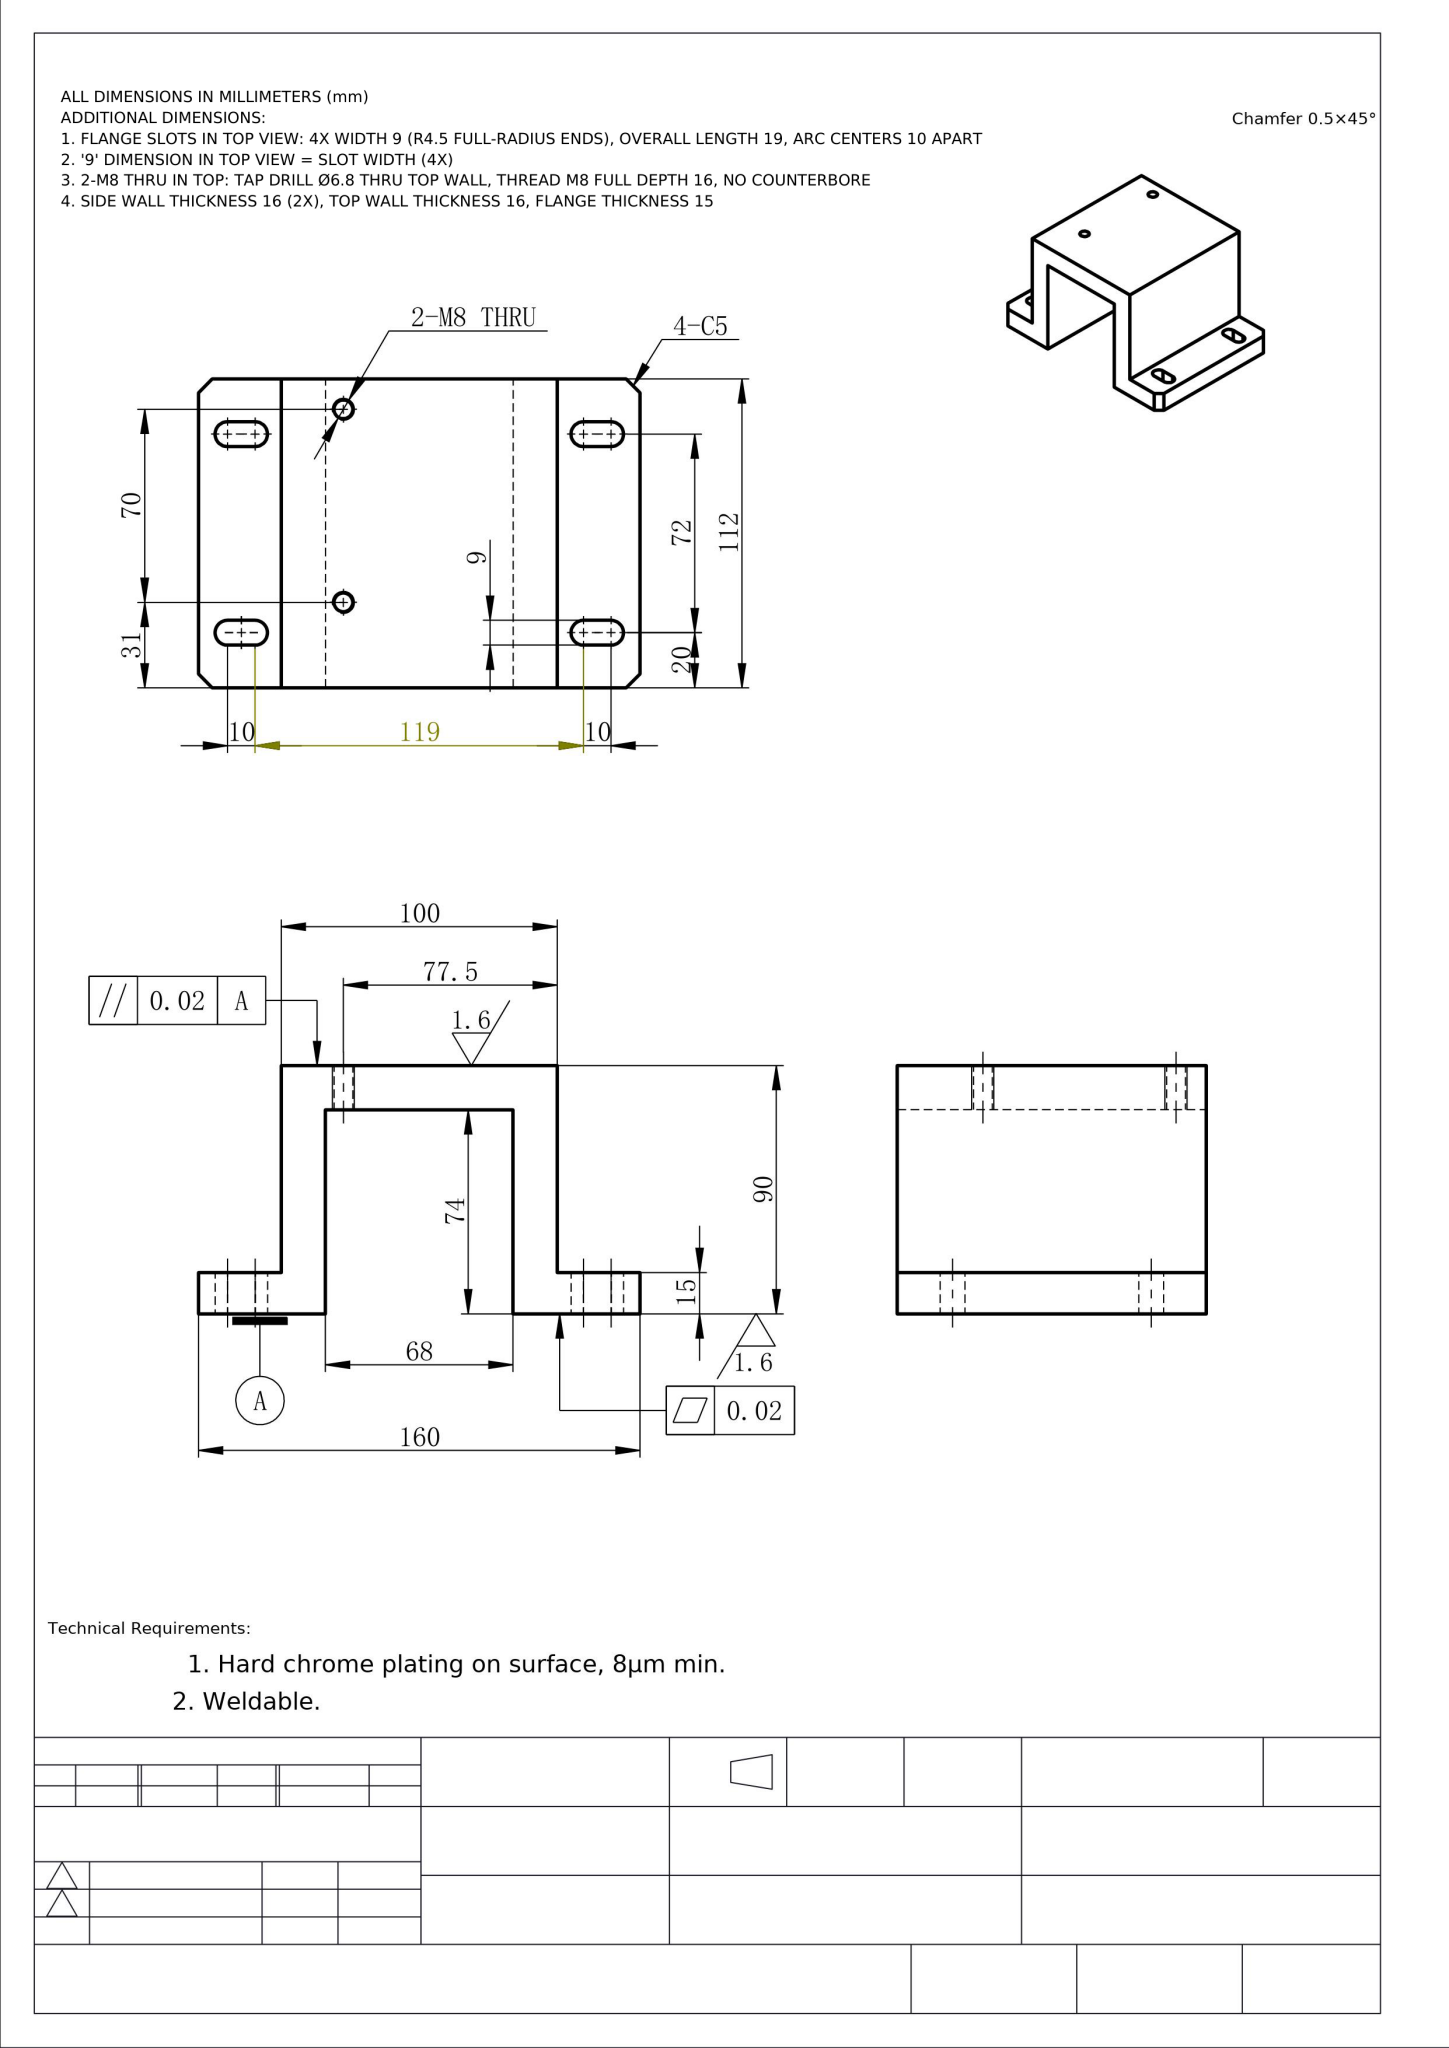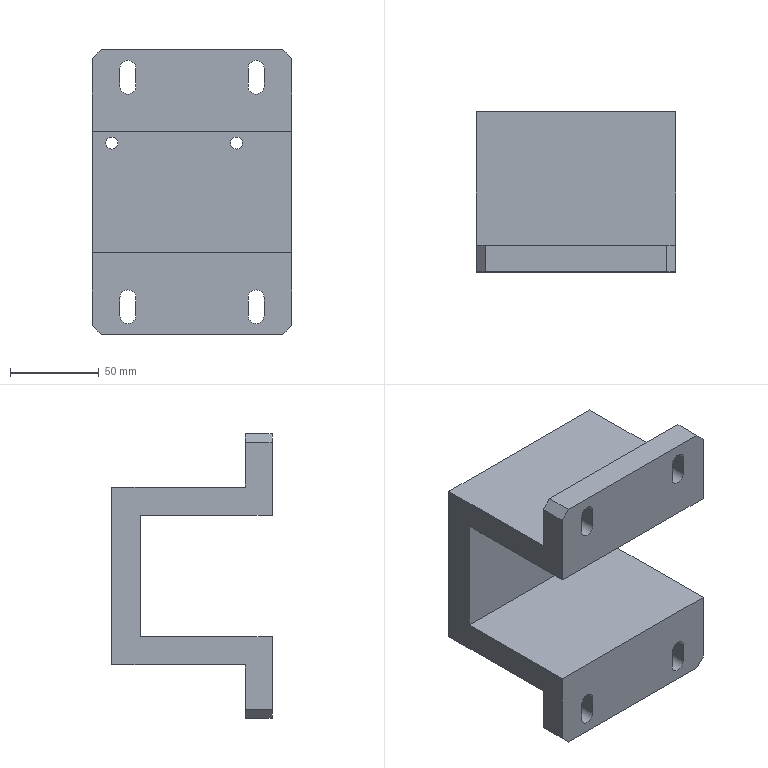Part | NX | mm | 1 solid | 42 faces | box 112 x 90 x 160 mm | volume 534087 mm3 | plane 26 | cylinder 16 | commonest cylinder face diameters 9 x12 6.8 x4